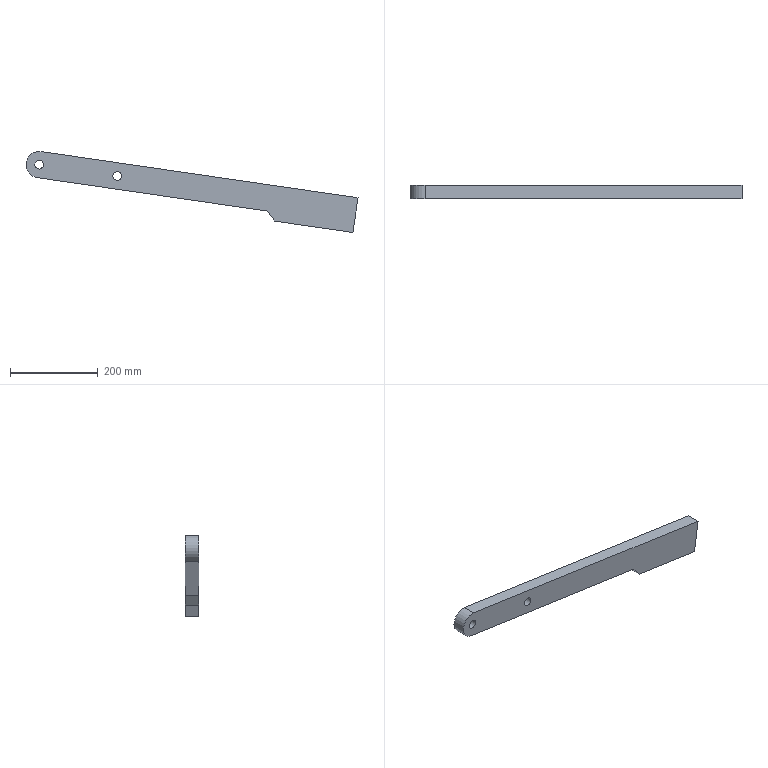Component | NX | POWER_ROD | 1 solid | 10 faces | box 756.72 x 30 x 184.54 mm | volume 1451562 mm3 | plane 7 | cylinder 3 | commonest cylinder face diameters 20 x2 60 x1
STEP:
#1=CARTESIAN_POINT('',(0.,0.,0.));
#2=DIRECTION('',(0.,0.,1.));
#3=DIRECTION('',(1.,0.,0.));
#4=AXIS2_PLACEMENT_3D('',#1,#2,#3);
#5=CARTESIAN_POINT('',(-229.318,-15.,366.158));
#6=VERTEX_POINT('',#5);
#7=CARTESIAN_POINT('',(-220.682,-15.,425.533));
#8=VERTEX_POINT('',#7);
#9=CARTESIAN_POINT('',(-225.,-15.,395.845));
#10=DIRECTION('',(0.,1.,0.));
#11=DIRECTION('',(0.9896,0.,-0.1439));
#12=AXIS2_PLACEMENT_3D('',#9,#10,#11);
#13=CIRCLE('',#12,30.);
#14=CARTESIAN_POINT('',(-225.,15.,395.845));
#15=DIRECTION('',(0.,-1.,0.));
#16=DIRECTION('',(-0.9896,0.,0.1439));
#17=AXIS2_PLACEMENT_3D('',#14,#15,#16);
#18=CYLINDRICAL_SURFACE('',#17,30.);
#19=CARTESIAN_POINT('',(9.425,30.));
#20=DIRECTION('',(-1.,0.));
#21=VECTOR('',#20,1.);
#22=LINE('',#19,#21);
#23=(GEOMETRIC_REPRESENTATION_CONTEXT(2)PARAMETRIC_REPRESENTATION_CONTEXT()REPRESENTATION_CONTEXT('',''));
#24=DEFINITIONAL_REPRESENTATION('',(#22),#23);
#25=PCURVE('',#18,#24);
#26=CARTESIAN_POINT('',(-225.,-15.,395.845));
#27=DIRECTION('',(0.,1.,0.));
#28=DIRECTION('',(0.9896,0.,-0.1439));
#29=AXIS2_PLACEMENT_3D('',#26,#27,#28);
#30=PLANE('',#29);
#31=CARTESIAN_POINT('',(0.,0.));
#32=DIRECTION('',(1.,-0.));
#33=AXIS2_PLACEMENT_2D('',#31,#32);
#34=CIRCLE('',#33,30.);
#35=(GEOMETRIC_REPRESENTATION_CONTEXT(2)PARAMETRIC_REPRESENTATION_CONTEXT()REPRESENTATION_CONTEXT('',''));
#36=DEFINITIONAL_REPRESENTATION('',(#34),#35);
#37=PCURVE('',#30,#36);
#38=SURFACE_CURVE('',#13,(#25,#37),.PCURVE_S1.);
#39=EDGE_CURVE('',#6,#8,#38,.T.);
#40=ORIENTED_EDGE('',*,*,#39,.T.);
#41=CARTESIAN_POINT('',(-220.682,15.,425.533));
#42=VERTEX_POINT('',#41);
#43=CARTESIAN_POINT('',(-220.682,15.,425.533));
#44=DIRECTION('',(0.,-1.,0.));
#45=VECTOR('',#44,1.);
#46=LINE('',#43,#45);
#47=CARTESIAN_POINT('',(4.712,0.));
#48=DIRECTION('',(0.,1.));
#49=VECTOR('',#48,1.);
#50=LINE('',#47,#49);
#51=(GEOMETRIC_REPRESENTATION_CONTEXT(2)PARAMETRIC_REPRESENTATION_CONTEXT()REPRESENTATION_CONTEXT('',''));
#52=DEFINITIONAL_REPRESENTATION('',(#50),#51);
#53=PCURVE('',#18,#52);
#54=CARTESIAN_POINT('',(274.112,15.,353.571));
#55=DIRECTION('',(-0.1439,0.,-0.9896));
#56=DIRECTION('',(-0.9896,0.,0.1439));
#57=AXIS2_PLACEMENT_3D('',#54,#55,#56);
#58=PLANE('',#57);
#59=CARTESIAN_POINT('',(500.,0.));
#60=DIRECTION('',(0.,-1.));
#61=VECTOR('',#60,1.);
#62=LINE('',#59,#61);
#63=(GEOMETRIC_REPRESENTATION_CONTEXT(2)PARAMETRIC_REPRESENTATION_CONTEXT()REPRESENTATION_CONTEXT('',''));
#64=DEFINITIONAL_REPRESENTATION('',(#62),#63);
#65=PCURVE('',#58,#64);
#66=SURFACE_CURVE('',#46,(#53,#65),.PCURVE_S1.);
#67=EDGE_CURVE('',#42,#8,#66,.T.);
#68=ORIENTED_EDGE('',*,*,#67,.F.);
#69=CARTESIAN_POINT('',(-229.318,15.,366.158));
#70=VERTEX_POINT('',#69);
#71=CARTESIAN_POINT('',(-225.,15.,395.845));
#72=DIRECTION('',(0.,1.,0.));
#73=DIRECTION('',(0.9896,0.,-0.1439));
#74=AXIS2_PLACEMENT_3D('',#71,#72,#73);
#75=CIRCLE('',#74,30.);
#76=CARTESIAN_POINT('',(9.425,0.));
#77=DIRECTION('',(-1.,0.));
#78=VECTOR('',#77,1.);
#79=LINE('',#76,#78);
#80=(GEOMETRIC_REPRESENTATION_CONTEXT(2)PARAMETRIC_REPRESENTATION_CONTEXT()REPRESENTATION_CONTEXT('',''));
#81=DEFINITIONAL_REPRESENTATION('',(#79),#80);
#82=PCURVE('',#18,#81);
#83=CARTESIAN_POINT('',(-225.,15.,395.845));
#84=DIRECTION('',(0.,1.,0.));
#85=DIRECTION('',(0.9896,0.,-0.1439));
#86=AXIS2_PLACEMENT_3D('',#83,#84,#85);
#87=PLANE('',#86);
#88=CARTESIAN_POINT('',(0.,0.));
#89=DIRECTION('',(1.,-0.));
#90=AXIS2_PLACEMENT_2D('',#88,#89);
#91=CIRCLE('',#90,30.);
#92=(GEOMETRIC_REPRESENTATION_CONTEXT(2)PARAMETRIC_REPRESENTATION_CONTEXT()REPRESENTATION_CONTEXT('',''));
#93=DEFINITIONAL_REPRESENTATION('',(#91),#92);
#94=PCURVE('',#87,#93);
#95=SURFACE_CURVE('',#75,(#82,#94),.PCURVE_S1.);
#96=EDGE_CURVE('',#70,#42,#95,.T.);
#97=ORIENTED_EDGE('',*,*,#96,.F.);
#98=CARTESIAN_POINT('',(-229.318,15.,366.158));
#99=DIRECTION('',(0.,-1.,0.));
#100=VECTOR('',#99,1.);
#101=LINE('',#98,#100);
#102=CARTESIAN_POINT('',(7.854,0.));
#103=DIRECTION('',(0.,1.));
#104=VECTOR('',#103,1.);
#105=LINE('',#102,#104);
#106=(GEOMETRIC_REPRESENTATION_CONTEXT(2)PARAMETRIC_REPRESENTATION_CONTEXT()REPRESENTATION_CONTEXT('',''));
#107=DEFINITIONAL_REPRESENTATION('',(#105),#106);
#108=PCURVE('',#18,#107);
#109=CARTESIAN_POINT('',(295.164,15.,289.878));
#110=DIRECTION('',(0.1439,0.,0.9896));
#111=DIRECTION('',(0.9896,0.,-0.1439));
#112=AXIS2_PLACEMENT_3D('',#109,#110,#111);
#113=PLANE('',#112);
#114=CARTESIAN_POINT('',(-530.,0.));
#115=DIRECTION('',(0.,-1.));
#116=VECTOR('',#115,1.);
#117=LINE('',#114,#116);
#118=(GEOMETRIC_REPRESENTATION_CONTEXT(2)PARAMETRIC_REPRESENTATION_CONTEXT()REPRESENTATION_CONTEXT('',''));
#119=DEFINITIONAL_REPRESENTATION('',(#117),#118);
#120=PCURVE('',#113,#119);
#121=SURFACE_CURVE('',#101,(#108,#120),.PCURVE_S1.);
#122=EDGE_CURVE('',#70,#6,#121,.T.);
#123=ORIENTED_EDGE('',*,*,#122,.T.);
#124=EDGE_LOOP('',(#40,#68,#97,#123));
#125=FACE_BOUND('',#124,.T.);
#126=ADVANCED_FACE('',(#125),#18,.T.);
#127=CARTESIAN_POINT('',(501.717,-15.,320.468));
#128=VERTEX_POINT('',#127);
#129=CARTESIAN_POINT('',(274.112,-15.,353.571));
#130=DIRECTION('',(0.9896,0.,-0.1439));
#131=VECTOR('',#130,1.);
#132=LINE('',#129,#131);
#133=CARTESIAN_POINT('',(0.,-30.));
#134=DIRECTION('',(-1.,0.));
#135=VECTOR('',#134,1.);
#136=LINE('',#133,#135);
#137=(GEOMETRIC_REPRESENTATION_CONTEXT(2)PARAMETRIC_REPRESENTATION_CONTEXT()REPRESENTATION_CONTEXT('',''));
#138=DEFINITIONAL_REPRESENTATION('',(#136),#137);
#139=PCURVE('',#58,#138);
#140=CARTESIAN_POINT('',(500.,-30.));
#141=DIRECTION('',(1.,0.));
#142=VECTOR('',#141,1.);
#143=LINE('',#140,#142);
#144=(GEOMETRIC_REPRESENTATION_CONTEXT(2)PARAMETRIC_REPRESENTATION_CONTEXT()REPRESENTATION_CONTEXT('',''));
#145=DEFINITIONAL_REPRESENTATION('',(#143),#144);
#146=PCURVE('',#30,#145);
#147=SURFACE_CURVE('',#132,(#139,#146),.PCURVE_S1.);
#148=EDGE_CURVE('',#8,#128,#147,.T.);
#149=ORIENTED_EDGE('',*,*,#148,.T.);
#150=CARTESIAN_POINT('',(501.717,15.,320.468));
#151=VERTEX_POINT('',#150);
#152=CARTESIAN_POINT('',(501.717,15.,320.468));
#153=DIRECTION('',(0.,-1.,0.));
#154=VECTOR('',#153,1.);
#155=LINE('',#152,#154);
#156=CARTESIAN_POINT('',(-230.,0.));
#157=DIRECTION('',(0.,-1.));
#158=VECTOR('',#157,1.);
#159=LINE('',#156,#158);
#160=(GEOMETRIC_REPRESENTATION_CONTEXT(2)PARAMETRIC_REPRESENTATION_CONTEXT()REPRESENTATION_CONTEXT('',''));
#161=DEFINITIONAL_REPRESENTATION('',(#159),#160);
#162=PCURVE('',#58,#161);
#163=CARTESIAN_POINT('',(501.717,15.,320.468));
#164=DIRECTION('',(-0.9896,0.,0.1439));
#165=DIRECTION('',(0.,1.,0.));
#166=AXIS2_PLACEMENT_3D('',#163,#164,#165);
#167=PLANE('',#166);
#168=CARTESIAN_POINT('',(0.,0.));
#169=DIRECTION('',(-1.,0.));
#170=VECTOR('',#169,1.);
#171=LINE('',#168,#170);
#172=(GEOMETRIC_REPRESENTATION_CONTEXT(2)PARAMETRIC_REPRESENTATION_CONTEXT()REPRESENTATION_CONTEXT('',''));
#173=DEFINITIONAL_REPRESENTATION('',(#171),#172);
#174=PCURVE('',#167,#173);
#175=SURFACE_CURVE('',#155,(#162,#174),.PCURVE_S1.);
#176=EDGE_CURVE('',#151,#128,#175,.T.);
#177=ORIENTED_EDGE('',*,*,#176,.F.);
#178=CARTESIAN_POINT('',(-220.682,15.,425.533));
#179=DIRECTION('',(0.9896,0.,-0.1439));
#180=VECTOR('',#179,1.);
#181=LINE('',#178,#180);
#182=CARTESIAN_POINT('',(500.,0.));
#183=DIRECTION('',(-1.,0.));
#184=VECTOR('',#183,1.);
#185=LINE('',#182,#184);
#186=(GEOMETRIC_REPRESENTATION_CONTEXT(2)PARAMETRIC_REPRESENTATION_CONTEXT()REPRESENTATION_CONTEXT('',''));
#187=DEFINITIONAL_REPRESENTATION('',(#185),#186);
#188=PCURVE('',#58,#187);
#189=CARTESIAN_POINT('',(0.,-30.));
#190=DIRECTION('',(1.,0.));
#191=VECTOR('',#190,1.);
#192=LINE('',#189,#191);
#193=(GEOMETRIC_REPRESENTATION_CONTEXT(2)PARAMETRIC_REPRESENTATION_CONTEXT()REPRESENTATION_CONTEXT('',''));
#194=DEFINITIONAL_REPRESENTATION('',(#192),#193);
#195=PCURVE('',#87,#194);
#196=SURFACE_CURVE('',#181,(#188,#195),.PCURVE_S1.);
#197=EDGE_CURVE('',#42,#151,#196,.T.);
#198=ORIENTED_EDGE('',*,*,#197,.F.);
#199=ORIENTED_EDGE('',*,*,#67,.T.);
#200=EDGE_LOOP('',(#149,#177,#198,#199));
#201=FACE_BOUND('',#200,.T.);
#202=ADVANCED_FACE('',(#201),#58,.F.);
#203=CARTESIAN_POINT('',(490.203,-15.,241.301));
#204=VERTEX_POINT('',#203);
#205=CARTESIAN_POINT('',(501.717,-15.,320.468));
#206=DIRECTION('',(-0.1439,0.,-0.9896));
#207=VECTOR('',#206,1.);
#208=LINE('',#205,#207);
#209=CARTESIAN_POINT('',(-30.,0.));
#210=DIRECTION('',(0.,1.));
#211=VECTOR('',#210,1.);
#212=LINE('',#209,#211);
#213=(GEOMETRIC_REPRESENTATION_CONTEXT(2)PARAMETRIC_REPRESENTATION_CONTEXT()REPRESENTATION_CONTEXT('',''));
#214=DEFINITIONAL_REPRESENTATION('',(#212),#213);
#215=PCURVE('',#167,#214);
#216=CARTESIAN_POINT('',(730.,-30.));
#217=DIRECTION('',(0.,1.));
#218=VECTOR('',#217,1.);
#219=LINE('',#216,#218);
#220=(GEOMETRIC_REPRESENTATION_CONTEXT(2)PARAMETRIC_REPRESENTATION_CONTEXT()REPRESENTATION_CONTEXT('',''));
#221=DEFINITIONAL_REPRESENTATION('',(#219),#220);
#222=PCURVE('',#30,#221);
#223=SURFACE_CURVE('',#208,(#215,#222),.PCURVE_S1.);
#224=EDGE_CURVE('',#128,#204,#223,.T.);
#225=ORIENTED_EDGE('',*,*,#224,.T.);
#226=CARTESIAN_POINT('',(490.203,15.,241.301));
#227=VERTEX_POINT('',#226);
#228=CARTESIAN_POINT('',(490.203,15.,241.301));
#229=DIRECTION('',(0.,-1.,0.));
#230=VECTOR('',#229,1.);
#231=LINE('',#228,#230);
#232=CARTESIAN_POINT('',(0.,80.));
#233=DIRECTION('',(-1.,0.));
#234=VECTOR('',#233,1.);
#235=LINE('',#232,#234);
#236=(GEOMETRIC_REPRESENTATION_CONTEXT(2)PARAMETRIC_REPRESENTATION_CONTEXT()REPRESENTATION_CONTEXT('',''));
#237=DEFINITIONAL_REPRESENTATION('',(#235),#236);
#238=PCURVE('',#167,#237);
#239=CARTESIAN_POINT('',(490.203,15.,241.301));
#240=DIRECTION('',(0.1439,0.,0.9896));
#241=DIRECTION('',(0.,-1.,0.));
#242=AXIS2_PLACEMENT_3D('',#239,#240,#241);
#243=PLANE('',#242);
#244=CARTESIAN_POINT('',(0.,0.));
#245=DIRECTION('',(1.,0.));
#246=VECTOR('',#245,1.);
#247=LINE('',#244,#246);
#248=(GEOMETRIC_REPRESENTATION_CONTEXT(2)PARAMETRIC_REPRESENTATION_CONTEXT()REPRESENTATION_CONTEXT('',''));
#249=DEFINITIONAL_REPRESENTATION('',(#247),#248);
#250=PCURVE('',#243,#249);
#251=SURFACE_CURVE('',#231,(#238,#250),.PCURVE_S1.);
#252=EDGE_CURVE('',#227,#204,#251,.T.);
#253=ORIENTED_EDGE('',*,*,#252,.F.);
#254=CARTESIAN_POINT('',(501.717,15.,320.468));
#255=DIRECTION('',(-0.1439,0.,-0.9896));
#256=VECTOR('',#255,1.);
#257=LINE('',#254,#256);
#258=CARTESIAN_POINT('',(0.,0.));
#259=DIRECTION('',(0.,1.));
#260=VECTOR('',#259,1.);
#261=LINE('',#258,#260);
#262=(GEOMETRIC_REPRESENTATION_CONTEXT(2)PARAMETRIC_REPRESENTATION_CONTEXT()REPRESENTATION_CONTEXT('',''));
#263=DEFINITIONAL_REPRESENTATION('',(#261),#262);
#264=PCURVE('',#167,#263);
#265=CARTESIAN_POINT('',(730.,-30.));
#266=DIRECTION('',(0.,1.));
#267=VECTOR('',#266,1.);
#268=LINE('',#265,#267);
#269=(GEOMETRIC_REPRESENTATION_CONTEXT(2)PARAMETRIC_REPRESENTATION_CONTEXT()REPRESENTATION_CONTEXT('',''));
#270=DEFINITIONAL_REPRESENTATION('',(#268),#269);
#271=PCURVE('',#87,#270);
#272=SURFACE_CURVE('',#257,(#264,#271),.PCURVE_S1.);
#273=EDGE_CURVE('',#151,#227,#272,.T.);
#274=ORIENTED_EDGE('',*,*,#273,.F.);
#275=ORIENTED_EDGE('',*,*,#176,.T.);
#276=EDGE_LOOP('',(#225,#253,#274,#275));
#277=FACE_BOUND('',#276,.T.);
#278=ADVANCED_FACE('',(#277),#167,.F.);
#279=CARTESIAN_POINT('',(312.078,-15.,267.207));
#280=VERTEX_POINT('',#279);
#281=CARTESIAN_POINT('',(490.203,-15.,241.301));
#282=DIRECTION('',(-0.9896,0.,0.1439));
#283=VECTOR('',#282,1.);
#284=LINE('',#281,#283);
#285=CARTESIAN_POINT('',(30.,0.));
#286=DIRECTION('',(0.,-1.));
#287=VECTOR('',#286,1.);
#288=LINE('',#285,#287);
#289=(GEOMETRIC_REPRESENTATION_CONTEXT(2)PARAMETRIC_REPRESENTATION_CONTEXT()REPRESENTATION_CONTEXT('',''));
#290=DEFINITIONAL_REPRESENTATION('',(#288),#289);
#291=PCURVE('',#243,#290);
#292=CARTESIAN_POINT('',(730.,50.));
#293=DIRECTION('',(-1.,0.));
#294=VECTOR('',#293,1.);
#295=LINE('',#292,#294);
#296=(GEOMETRIC_REPRESENTATION_CONTEXT(2)PARAMETRIC_REPRESENTATION_CONTEXT()REPRESENTATION_CONTEXT('',''));
#297=DEFINITIONAL_REPRESENTATION('',(#295),#296);
#298=PCURVE('',#30,#297);
#299=SURFACE_CURVE('',#284,(#291,#298),.PCURVE_S1.);
#300=EDGE_CURVE('',#204,#280,#299,.T.);
#301=ORIENTED_EDGE('',*,*,#300,.T.);
#302=CARTESIAN_POINT('',(312.078,15.,267.207));
#303=VERTEX_POINT('',#302);
#304=CARTESIAN_POINT('',(312.078,15.,267.207));
#305=DIRECTION('',(0.,-1.,0.));
#306=VECTOR('',#305,1.);
#307=LINE('',#304,#306);
#308=CARTESIAN_POINT('',(0.,-180.));
#309=DIRECTION('',(1.,0.));
#310=VECTOR('',#309,1.);
#311=LINE('',#308,#310);
#312=(GEOMETRIC_REPRESENTATION_CONTEXT(2)PARAMETRIC_REPRESENTATION_CONTEXT()REPRESENTATION_CONTEXT('',''));
#313=DEFINITIONAL_REPRESENTATION('',(#311),#312);
#314=PCURVE('',#243,#313);
#315=CARTESIAN_POINT('',(312.078,15.,267.207));
#316=DIRECTION('',(0.8015,0.,0.598));
#317=DIRECTION('',(0.598,0.,-0.8015));
#318=AXIS2_PLACEMENT_3D('',#315,#316,#317);
#319=PLANE('',#318);
#320=CARTESIAN_POINT('',(0.,0.));
#321=DIRECTION('',(0.,-1.));
#322=VECTOR('',#321,1.);
#323=LINE('',#320,#322);
#324=(GEOMETRIC_REPRESENTATION_CONTEXT(2)PARAMETRIC_REPRESENTATION_CONTEXT()REPRESENTATION_CONTEXT('',''));
#325=DEFINITIONAL_REPRESENTATION('',(#323),#324);
#326=PCURVE('',#319,#325);
#327=SURFACE_CURVE('',#307,(#314,#326),.PCURVE_S1.);
#328=EDGE_CURVE('',#303,#280,#327,.T.);
#329=ORIENTED_EDGE('',*,*,#328,.F.);
#330=CARTESIAN_POINT('',(490.203,15.,241.301));
#331=DIRECTION('',(-0.9896,0.,0.1439));
#332=VECTOR('',#331,1.);
#333=LINE('',#330,#332);
#334=CARTESIAN_POINT('',(0.,0.));
#335=DIRECTION('',(0.,-1.));
#336=VECTOR('',#335,1.);
#337=LINE('',#334,#336);
#338=(GEOMETRIC_REPRESENTATION_CONTEXT(2)PARAMETRIC_REPRESENTATION_CONTEXT()REPRESENTATION_CONTEXT('',''));
#339=DEFINITIONAL_REPRESENTATION('',(#337),#338);
#340=PCURVE('',#243,#339);
#341=CARTESIAN_POINT('',(730.,50.));
#342=DIRECTION('',(-1.,0.));
#343=VECTOR('',#342,1.);
#344=LINE('',#341,#343);
#345=(GEOMETRIC_REPRESENTATION_CONTEXT(2)PARAMETRIC_REPRESENTATION_CONTEXT()REPRESENTATION_CONTEXT('',''));
#346=DEFINITIONAL_REPRESENTATION('',(#344),#345);
#347=PCURVE('',#87,#346);
#348=SURFACE_CURVE('',#333,(#340,#347),.PCURVE_S1.);
#349=EDGE_CURVE('',#227,#303,#348,.T.);
#350=ORIENTED_EDGE('',*,*,#349,.F.);
#351=ORIENTED_EDGE('',*,*,#252,.T.);
#352=EDGE_LOOP('',(#301,#329,#350,#351));
#353=FACE_BOUND('',#352,.T.);
#354=ADVANCED_FACE('',(#353),#243,.F.);
#355=CARTESIAN_POINT('',(295.164,-15.,289.878));
#356=VERTEX_POINT('',#355);
#357=CARTESIAN_POINT('',(312.078,-15.,267.207));
#358=DIRECTION('',(-0.598,0.,0.8015));
#359=VECTOR('',#358,1.);
#360=LINE('',#357,#359);
#361=CARTESIAN_POINT('',(0.,-30.));
#362=DIRECTION('',(-1.,0.));
#363=VECTOR('',#362,1.);
#364=LINE('',#361,#363);
#365=(GEOMETRIC_REPRESENTATION_CONTEXT(2)PARAMETRIC_REPRESENTATION_CONTEXT()REPRESENTATION_CONTEXT('',''));
#366=DEFINITIONAL_REPRESENTATION('',(#364),#365);
#367=PCURVE('',#319,#366);
#368=CARTESIAN_POINT('',(550.,50.));
#369=DIRECTION('',(-0.7071,-0.7071));
#370=VECTOR('',#369,1.);
#371=LINE('',#368,#370);
#372=(GEOMETRIC_REPRESENTATION_CONTEXT(2)PARAMETRIC_REPRESENTATION_CONTEXT()REPRESENTATION_CONTEXT('',''));
#373=DEFINITIONAL_REPRESENTATION('',(#371),#372);
#374=PCURVE('',#30,#373);
#375=SURFACE_CURVE('',#360,(#367,#374),.PCURVE_S1.);
#376=EDGE_CURVE('',#280,#356,#375,.T.);
#377=ORIENTED_EDGE('',*,*,#376,.T.);
#378=CARTESIAN_POINT('',(295.164,15.,289.878));
#379=VERTEX_POINT('',#378);
#380=CARTESIAN_POINT('',(295.164,15.,289.878));
#381=DIRECTION('',(0.,-1.,0.));
#382=VECTOR('',#381,1.);
#383=LINE('',#380,#382);
#384=CARTESIAN_POINT('',(-28.284,0.));
#385=DIRECTION('',(0.,-1.));
#386=VECTOR('',#385,1.);
#387=LINE('',#384,#386);
#388=(GEOMETRIC_REPRESENTATION_CONTEXT(2)PARAMETRIC_REPRESENTATION_CONTEXT()REPRESENTATION_CONTEXT('',''));
#389=DEFINITIONAL_REPRESENTATION('',(#387),#388);
#390=PCURVE('',#319,#389);
#391=CARTESIAN_POINT('',(0.,0.));
#392=DIRECTION('',(0.,-1.));
#393=VECTOR('',#392,1.);
#394=LINE('',#391,#393);
#395=(GEOMETRIC_REPRESENTATION_CONTEXT(2)PARAMETRIC_REPRESENTATION_CONTEXT()REPRESENTATION_CONTEXT('',''));
#396=DEFINITIONAL_REPRESENTATION('',(#394),#395);
#397=PCURVE('',#113,#396);
#398=SURFACE_CURVE('',#383,(#390,#397),.PCURVE_S1.);
#399=EDGE_CURVE('',#379,#356,#398,.T.);
#400=ORIENTED_EDGE('',*,*,#399,.F.);
#401=CARTESIAN_POINT('',(312.078,15.,267.207));
#402=DIRECTION('',(-0.598,0.,0.8015));
#403=VECTOR('',#402,1.);
#404=LINE('',#401,#403);
#405=CARTESIAN_POINT('',(0.,0.));
#406=DIRECTION('',(-1.,0.));
#407=VECTOR('',#406,1.);
#408=LINE('',#405,#407);
#409=(GEOMETRIC_REPRESENTATION_CONTEXT(2)PARAMETRIC_REPRESENTATION_CONTEXT()REPRESENTATION_CONTEXT('',''));
#410=DEFINITIONAL_REPRESENTATION('',(#408),#409);
#411=PCURVE('',#319,#410);
#412=CARTESIAN_POINT('',(550.,50.));
#413=DIRECTION('',(-0.7071,-0.7071));
#414=VECTOR('',#413,1.);
#415=LINE('',#412,#414);
#416=(GEOMETRIC_REPRESENTATION_CONTEXT(2)PARAMETRIC_REPRESENTATION_CONTEXT()REPRESENTATION_CONTEXT('',''));
#417=DEFINITIONAL_REPRESENTATION('',(#415),#416);
#418=PCURVE('',#87,#417);
#419=SURFACE_CURVE('',#404,(#411,#418),.PCURVE_S1.);
#420=EDGE_CURVE('',#303,#379,#419,.T.);
#421=ORIENTED_EDGE('',*,*,#420,.F.);
#422=ORIENTED_EDGE('',*,*,#328,.T.);
#423=EDGE_LOOP('',(#377,#400,#421,#422));
#424=FACE_BOUND('',#423,.T.);
#425=ADVANCED_FACE('',(#424),#319,.F.);
#426=CARTESIAN_POINT('',(-215.104,15.,394.406));
#427=VERTEX_POINT('',#426);
#428=CARTESIAN_POINT('',(-225.,15.,395.845));
#429=DIRECTION('',(0.,1.,0.));
#430=DIRECTION('',(0.9896,0.,-0.1439));
#431=AXIS2_PLACEMENT_3D('',#428,#429,#430);
#432=CIRCLE('',#431,10.);
#433=CARTESIAN_POINT('',(-225.,15.,395.845));
#434=DIRECTION('',(0.,-1.,0.));
#435=DIRECTION('',(-0.9896,0.,0.1439));
#436=AXIS2_PLACEMENT_3D('',#433,#434,#435);
#437=CYLINDRICAL_SURFACE('',#436,10.);
#438=CARTESIAN_POINT('',(9.425,0.));
#439=DIRECTION('',(-1.,0.));
#440=VECTOR('',#439,1.);
#441=LINE('',#438,#440);
#442=(GEOMETRIC_REPRESENTATION_CONTEXT(2)PARAMETRIC_REPRESENTATION_CONTEXT()REPRESENTATION_CONTEXT('',''));
#443=DEFINITIONAL_REPRESENTATION('',(#441),#442);
#444=PCURVE('',#437,#443);
#445=CARTESIAN_POINT('',(0.,0.));
#446=DIRECTION('',(1.,0.));
#447=AXIS2_PLACEMENT_2D('',#445,#446);
#448=CIRCLE('',#447,10.);
#449=(GEOMETRIC_REPRESENTATION_CONTEXT(2)PARAMETRIC_REPRESENTATION_CONTEXT()REPRESENTATION_CONTEXT('',''));
#450=DEFINITIONAL_REPRESENTATION('',(#448),#449);
#451=PCURVE('',#87,#450);
#452=SURFACE_CURVE('',#432,(#444,#451),.PCURVE_S1.);
#453=EDGE_CURVE('',#427,#427,#452,.T.);
#454=ORIENTED_EDGE('',*,*,#453,.F.);
#455=CARTESIAN_POINT('',(-215.104,-15.,394.406));
#456=VERTEX_POINT('',#455);
#457=CARTESIAN_POINT('',(-215.104,15.,394.406));
#458=CARTESIAN_POINT('',(-215.104,-15.,394.406));
#459=B_SPLINE_CURVE_WITH_KNOTS('',1,(#457,#458),.UNSPECIFIED.,.F.,.F.,(2,2),(0.,30.),.PIECEWISE_BEZIER_KNOTS.);
#460=CARTESIAN_POINT('',(9.425,0.));
#461=DIRECTION('',(0.,1.));
#462=VECTOR('',#461,1.);
#463=LINE('',#460,#462);
#464=(GEOMETRIC_REPRESENTATION_CONTEXT(2)PARAMETRIC_REPRESENTATION_CONTEXT()REPRESENTATION_CONTEXT('',''));
#465=DEFINITIONAL_REPRESENTATION('',(#463),#464);
#466=PCURVE('',#437,#465);
#467=CARTESIAN_POINT('',(3.142,0.));
#468=DIRECTION('',(0.,1.));
#469=VECTOR('',#468,1.);
#470=LINE('',#467,#469);
#471=(GEOMETRIC_REPRESENTATION_CONTEXT(2)PARAMETRIC_REPRESENTATION_CONTEXT()REPRESENTATION_CONTEXT('',''));
#472=DEFINITIONAL_REPRESENTATION('',(#470),#471);
#473=PCURVE('',#437,#472);
#474=SEAM_CURVE('',#459,(#466,#473),.PCURVE_S1.);
#475=EDGE_CURVE('',#427,#456,#474,.T.);
#476=ORIENTED_EDGE('',*,*,#475,.T.);
#477=CARTESIAN_POINT('',(-225.,-15.,395.845));
#478=DIRECTION('',(0.,1.,0.));
#479=DIRECTION('',(0.9896,0.,-0.1439));
#480=AXIS2_PLACEMENT_3D('',#477,#478,#479);
#481=CIRCLE('',#480,10.);
#482=CARTESIAN_POINT('',(9.425,30.));
#483=DIRECTION('',(-1.,0.));
#484=VECTOR('',#483,1.);
#485=LINE('',#482,#484);
#486=(GEOMETRIC_REPRESENTATION_CONTEXT(2)PARAMETRIC_REPRESENTATION_CONTEXT()REPRESENTATION_CONTEXT('',''));
#487=DEFINITIONAL_REPRESENTATION('',(#485),#486);
#488=PCURVE('',#437,#487);
#489=CARTESIAN_POINT('',(0.,0.));
#490=DIRECTION('',(1.,0.));
#491=AXIS2_PLACEMENT_2D('',#489,#490);
#492=CIRCLE('',#491,10.);
#493=(GEOMETRIC_REPRESENTATION_CONTEXT(2)PARAMETRIC_REPRESENTATION_CONTEXT()REPRESENTATION_CONTEXT('',''));
#494=DEFINITIONAL_REPRESENTATION('',(#492),#493);
#495=PCURVE('',#30,#494);
#496=SURFACE_CURVE('',#481,(#488,#495),.PCURVE_S1.);
#497=EDGE_CURVE('',#456,#456,#496,.T.);
#498=ORIENTED_EDGE('',*,*,#497,.T.);
#499=ORIENTED_EDGE('',*,*,#475,.F.);
#500=EDGE_LOOP('',(#454,#476,#498,#499));
#501=FACE_BOUND('',#500,.F.);
#502=ADVANCED_FACE('',(#501),#437,.F.);
#503=CARTESIAN_POINT('',(295.164,-15.,289.878));
#504=DIRECTION('',(-0.9896,0.,0.1439));
#505=VECTOR('',#504,1.);
#506=LINE('',#503,#505);
#507=CARTESIAN_POINT('',(0.,-30.));
#508=DIRECTION('',(-1.,0.));
#509=VECTOR('',#508,1.);
#510=LINE('',#507,#509);
#511=(GEOMETRIC_REPRESENTATION_CONTEXT(2)PARAMETRIC_REPRESENTATION_CONTEXT()REPRESENTATION_CONTEXT('',''));
#512=DEFINITIONAL_REPRESENTATION('',(#510),#511);
#513=PCURVE('',#113,#512);
#514=CARTESIAN_POINT('',(530.,30.));
#515=DIRECTION('',(-1.,0.));
#516=VECTOR('',#515,1.);
#517=LINE('',#514,#516);
#518=(GEOMETRIC_REPRESENTATION_CONTEXT(2)PARAMETRIC_REPRESENTATION_CONTEXT()REPRESENTATION_CONTEXT('',''));
#519=DEFINITIONAL_REPRESENTATION('',(#517),#518);
#520=PCURVE('',#30,#519);
#521=SURFACE_CURVE('',#506,(#513,#520),.PCURVE_S1.);
#522=EDGE_CURVE('',#356,#6,#521,.T.);
#523=ORIENTED_EDGE('',*,*,#522,.T.);
#524=ORIENTED_EDGE('',*,*,#122,.F.);
#525=CARTESIAN_POINT('',(295.164,15.,289.878));
#526=DIRECTION('',(-0.9896,0.,0.1439));
#527=VECTOR('',#526,1.);
#528=LINE('',#525,#527);
#529=CARTESIAN_POINT('',(0.,0.));
#530=DIRECTION('',(-1.,0.));
#531=VECTOR('',#530,1.);
#532=LINE('',#529,#531);
#533=(GEOMETRIC_REPRESENTATION_CONTEXT(2)PARAMETRIC_REPRESENTATION_CONTEXT()REPRESENTATION_CONTEXT('',''));
#534=DEFINITIONAL_REPRESENTATION('',(#532),#533);
#535=PCURVE('',#113,#534);
#536=CARTESIAN_POINT('',(530.,30.));
#537=DIRECTION('',(-1.,0.));
#538=VECTOR('',#537,1.);
#539=LINE('',#536,#538);
#540=(GEOMETRIC_REPRESENTATION_CONTEXT(2)PARAMETRIC_REPRESENTATION_CONTEXT()REPRESENTATION_CONTEXT('',''));
#541=DEFINITIONAL_REPRESENTATION('',(#539),#540);
#542=PCURVE('',#87,#541);
#543=SURFACE_CURVE('',#528,(#535,#542),.PCURVE_S1.);
#544=EDGE_CURVE('',#379,#70,#543,.T.);
#545=ORIENTED_EDGE('',*,*,#544,.F.);
#546=ORIENTED_EDGE('',*,*,#399,.T.);
#547=EDGE_LOOP('',(#523,#524,#545,#546));
#548=FACE_BOUND('',#547,.T.);
#549=ADVANCED_FACE('',(#548),#113,.F.);
#550=CARTESIAN_POINT('',(-36.978,15.,368.5));
#551=VERTEX_POINT('',#550);
#552=CARTESIAN_POINT('',(-46.874,15.,369.939));
#553=DIRECTION('',(0.,1.,0.));
#554=DIRECTION('',(0.9896,0.,-0.1439));
#555=AXIS2_PLACEMENT_3D('',#552,#553,#554);
#556=CIRCLE('',#555,10.);
#557=CARTESIAN_POINT('',(-46.874,15.,369.939));
#558=DIRECTION('',(0.,-1.,0.));
#559=DIRECTION('',(-0.9896,0.,0.1439));
#560=AXIS2_PLACEMENT_3D('',#557,#558,#559);
#561=CYLINDRICAL_SURFACE('',#560,10.);
#562=CARTESIAN_POINT('',(9.425,0.));
#563=DIRECTION('',(-1.,0.));
#564=VECTOR('',#563,1.);
#565=LINE('',#562,#564);
#566=(GEOMETRIC_REPRESENTATION_CONTEXT(2)PARAMETRIC_REPRESENTATION_CONTEXT()REPRESENTATION_CONTEXT('',''));
#567=DEFINITIONAL_REPRESENTATION('',(#565),#566);
#568=PCURVE('',#561,#567);
#569=CARTESIAN_POINT('',(180.,0.));
#570=DIRECTION('',(1.,0.));
#571=AXIS2_PLACEMENT_2D('',#569,#570);
#572=CIRCLE('',#571,10.);
#573=(GEOMETRIC_REPRESENTATION_CONTEXT(2)PARAMETRIC_REPRESENTATION_CONTEXT()REPRESENTATION_CONTEXT('',''));
#574=DEFINITIONAL_REPRESENTATION('',(#572),#573);
#575=PCURVE('',#87,#574);
#576=SURFACE_CURVE('',#556,(#568,#575),.PCURVE_S1.);
#577=EDGE_CURVE('',#551,#551,#576,.T.);
#578=ORIENTED_EDGE('',*,*,#577,.F.);
#579=CARTESIAN_POINT('',(-36.978,-15.,368.5));
#580=VERTEX_POINT('',#579);
#581=CARTESIAN_POINT('',(-36.978,15.,368.5));
#582=CARTESIAN_POINT('',(-36.978,-15.,368.5));
#583=B_SPLINE_CURVE_WITH_KNOTS('',1,(#581,#582),.UNSPECIFIED.,.F.,.F.,(2,2),(0.,30.),.PIECEWISE_BEZIER_KNOTS.);
#584=CARTESIAN_POINT('',(9.425,0.));
#585=DIRECTION('',(0.,1.));
#586=VECTOR('',#585,1.);
#587=LINE('',#584,#586);
#588=(GEOMETRIC_REPRESENTATION_CONTEXT(2)PARAMETRIC_REPRESENTATION_CONTEXT()REPRESENTATION_CONTEXT('',''));
#589=DEFINITIONAL_REPRESENTATION('',(#587),#588);
#590=PCURVE('',#561,#589);
#591=CARTESIAN_POINT('',(3.142,0.));
#592=DIRECTION('',(0.,1.));
#593=VECTOR('',#592,1.);
#594=LINE('',#591,#593);
#595=(GEOMETRIC_REPRESENTATION_CONTEXT(2)PARAMETRIC_REPRESENTATION_CONTEXT()REPRESENTATION_CONTEXT('',''));
#596=DEFINITIONAL_REPRESENTATION('',(#594),#595);
#597=PCURVE('',#561,#596);
#598=SEAM_CURVE('',#583,(#590,#597),.PCURVE_S1.);
#599=EDGE_CURVE('',#551,#580,#598,.T.);
#600=ORIENTED_EDGE('',*,*,#599,.T.);
#601=CARTESIAN_POINT('',(-46.874,-15.,369.939));
#602=DIRECTION('',(0.,1.,0.));
#603=DIRECTION('',(0.9896,0.,-0.1439));
#604=AXIS2_PLACEMENT_3D('',#601,#602,#603);
#605=CIRCLE('',#604,10.);
#606=CARTESIAN_POINT('',(9.425,30.));
#607=DIRECTION('',(-1.,0.));
#608=VECTOR('',#607,1.);
#609=LINE('',#606,#608);
#610=(GEOMETRIC_REPRESENTATION_CONTEXT(2)PARAMETRIC_REPRESENTATION_CONTEXT()REPRESENTATION_CONTEXT('',''));
#611=DEFINITIONAL_REPRESENTATION('',(#609),#610);
#612=PCURVE('',#561,#611);
#613=CARTESIAN_POINT('',(180.,0.));
#614=DIRECTION('',(1.,0.));
#615=AXIS2_PLACEMENT_2D('',#613,#614);
#616=CIRCLE('',#615,10.);
#617=(GEOMETRIC_REPRESENTATION_CONTEXT(2)PARAMETRIC_REPRESENTATION_CONTEXT()REPRESENTATION_CONTEXT('',''));
#618=DEFINITIONAL_REPRESENTATION('',(#616),#617);
#619=PCURVE('',#30,#618);
#620=SURFACE_CURVE('',#605,(#612,#619),.PCURVE_S1.);
#621=EDGE_CURVE('',#580,#580,#620,.T.);
#622=ORIENTED_EDGE('',*,*,#621,.T.);
#623=ORIENTED_EDGE('',*,*,#599,.F.);
#624=EDGE_LOOP('',(#578,#600,#622,#623));
#625=FACE_BOUND('',#624,.F.);
#626=ADVANCED_FACE('',(#625),#561,.F.);
#627=ORIENTED_EDGE('',*,*,#96,.T.);
#628=ORIENTED_EDGE('',*,*,#197,.T.);
#629=ORIENTED_EDGE('',*,*,#273,.T.);
#630=ORIENTED_EDGE('',*,*,#349,.T.);
#631=ORIENTED_EDGE('',*,*,#420,.T.);
#632=ORIENTED_EDGE('',*,*,#544,.T.);
#633=EDGE_LOOP('',(#627,#628,#629,#630,#631,#632));
#634=FACE_BOUND('',#633,.T.);
#635=ORIENTED_EDGE('',*,*,#453,.F.);
#636=EDGE_LOOP('',(#635));
#637=FACE_BOUND('',#636,.T.);
#638=ORIENTED_EDGE('',*,*,#577,.F.);
#639=EDGE_LOOP('',(#638));
#640=FACE_BOUND('',#639,.T.);
#641=ADVANCED_FACE('',(#634,#637,#640),#87,.T.);
#642=ORIENTED_EDGE('',*,*,#39,.F.);
#643=ORIENTED_EDGE('',*,*,#522,.F.);
#644=ORIENTED_EDGE('',*,*,#376,.F.);
#645=ORIENTED_EDGE('',*,*,#300,.F.);
#646=ORIENTED_EDGE('',*,*,#224,.F.);
#647=ORIENTED_EDGE('',*,*,#148,.F.);
#648=EDGE_LOOP('',(#642,#643,#644,#645,#646,#647));
#649=FACE_BOUND('',#648,.T.);
#650=ORIENTED_EDGE('',*,*,#497,.T.);
#651=EDGE_LOOP('',(#650));
#652=FACE_BOUND('',#651,.T.);
#653=ORIENTED_EDGE('',*,*,#621,.T.);
#654=EDGE_LOOP('',(#653));
#655=FACE_BOUND('',#654,.T.);
#656=ADVANCED_FACE('',(#649,#652,#655),#30,.F.);
#657=CLOSED_SHELL('',(#126,#202,#278,#354,#425,#502,#549,#626,#641,#656));
#658=MANIFOLD_SOLID_BREP('',#657);
#659=(LENGTH_UNIT()NAMED_UNIT(*)SI_UNIT(.MILLI.,.METRE.));
#660=UNCERTAINTY_MEASURE_WITH_UNIT(LENGTH_MEASURE(0.000002),#659,'','');
#661=(NAMED_UNIT(*)PLANE_ANGLE_UNIT()SI_UNIT($,.RADIAN.));
#662=(NAMED_UNIT(*)SI_UNIT($,.STERADIAN.)SOLID_ANGLE_UNIT());
#663=(GEOMETRIC_REPRESENTATION_CONTEXT(3)GLOBAL_UNCERTAINTY_ASSIGNED_CONTEXT((#660))GLOBAL_UNIT_ASSIGNED_CONTEXT((#659,#661,#662))REPRESENTATION_CONTEXT('',''));
#664=ADVANCED_BREP_SHAPE_REPRESENTATION('',(#4,#658),#663);